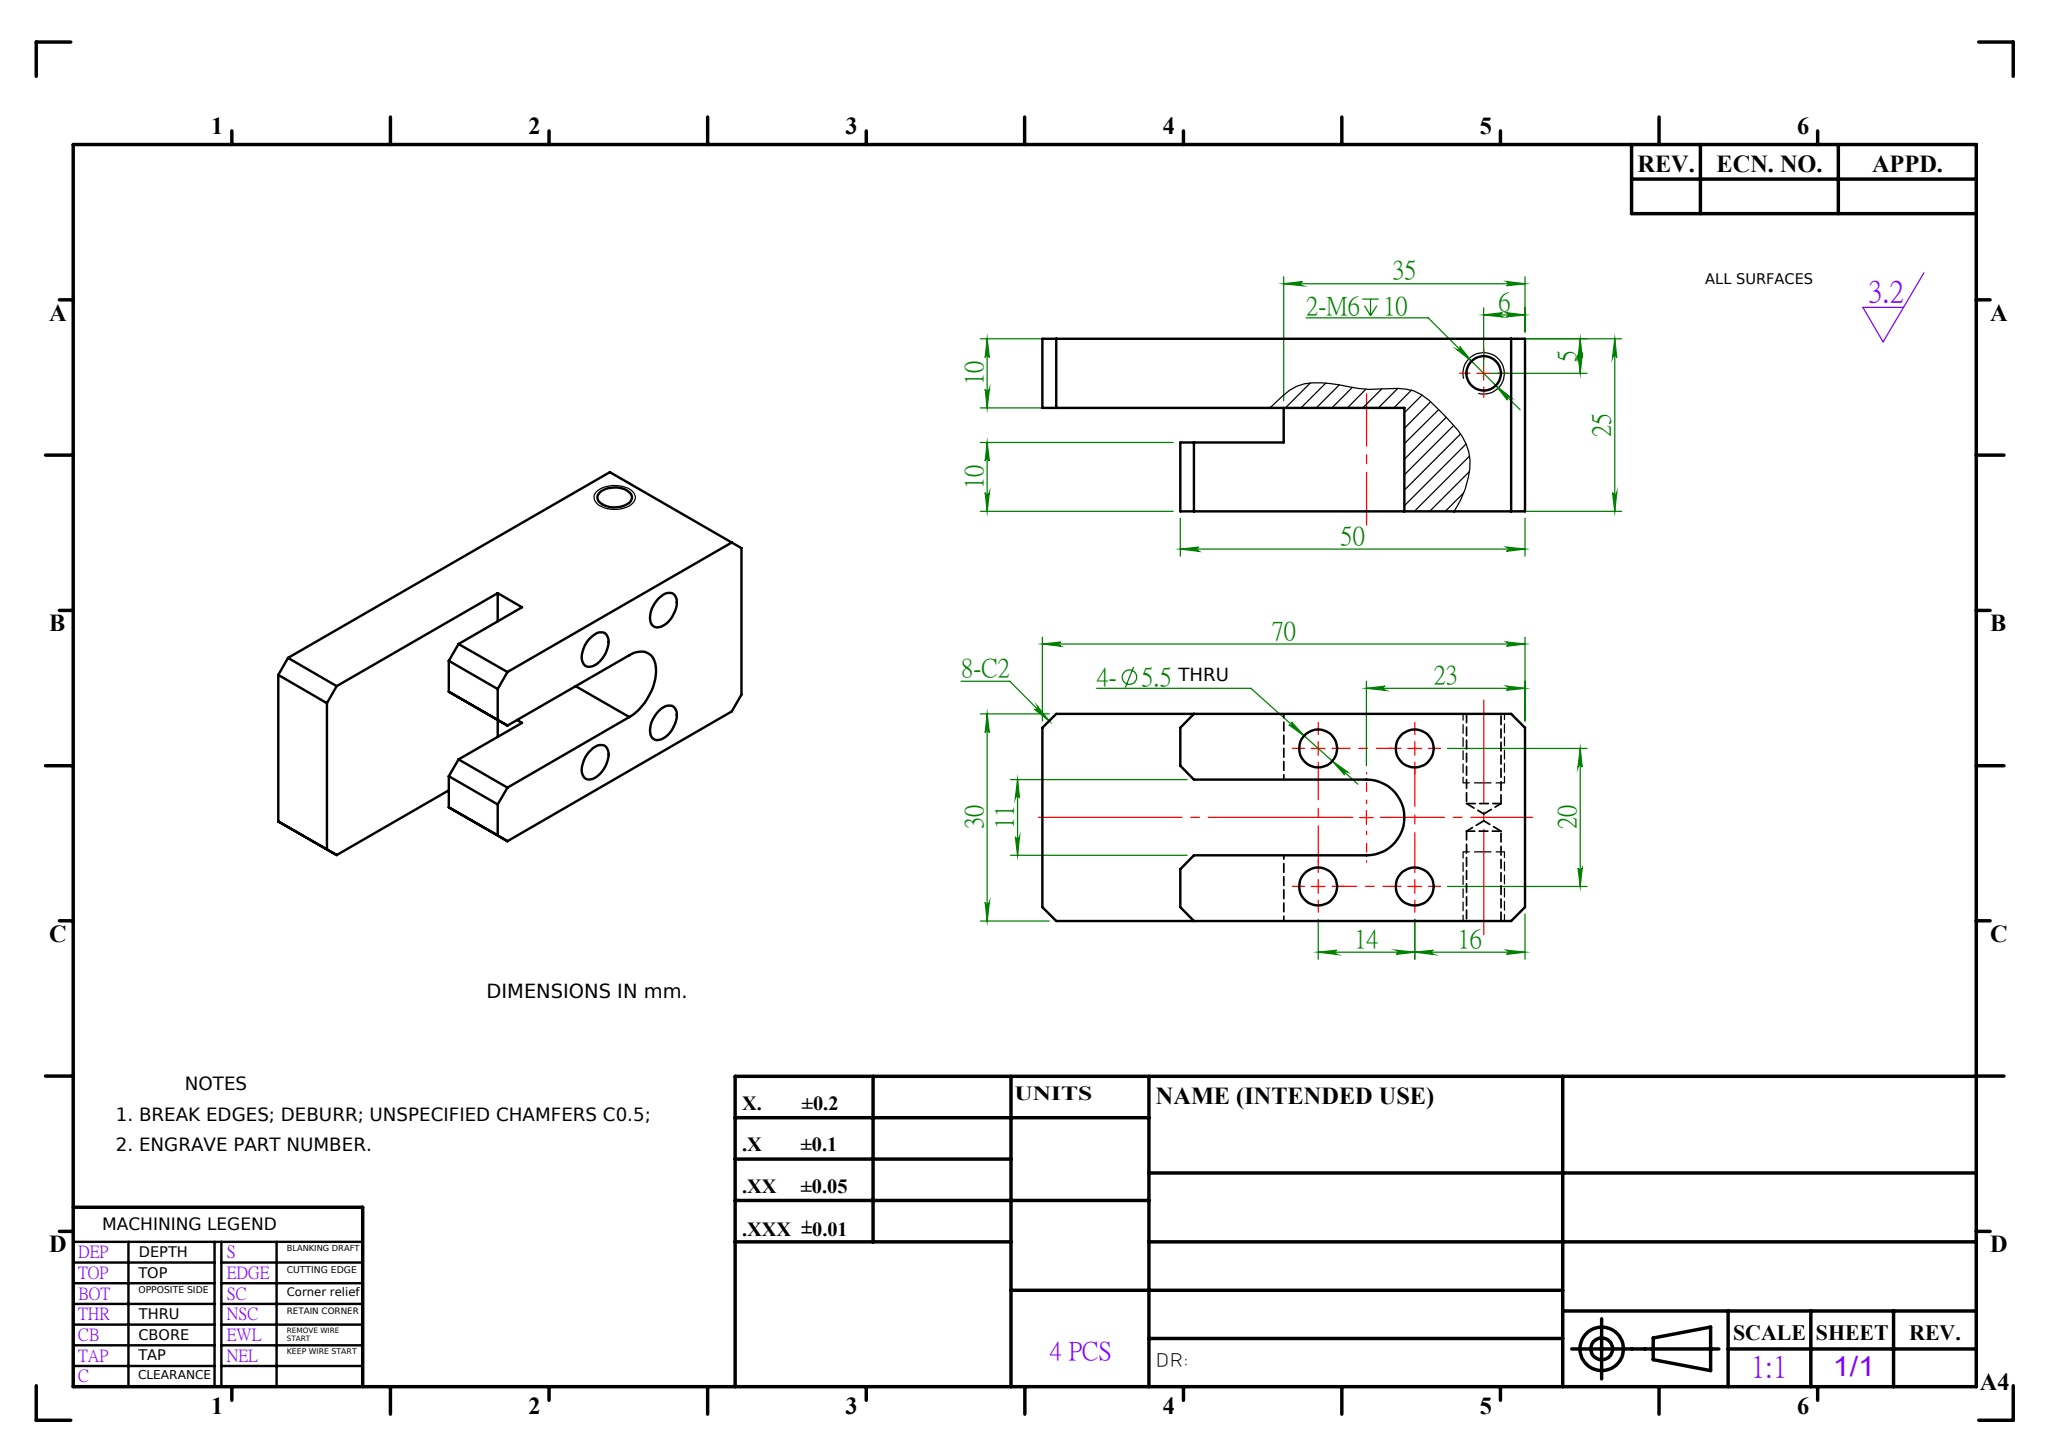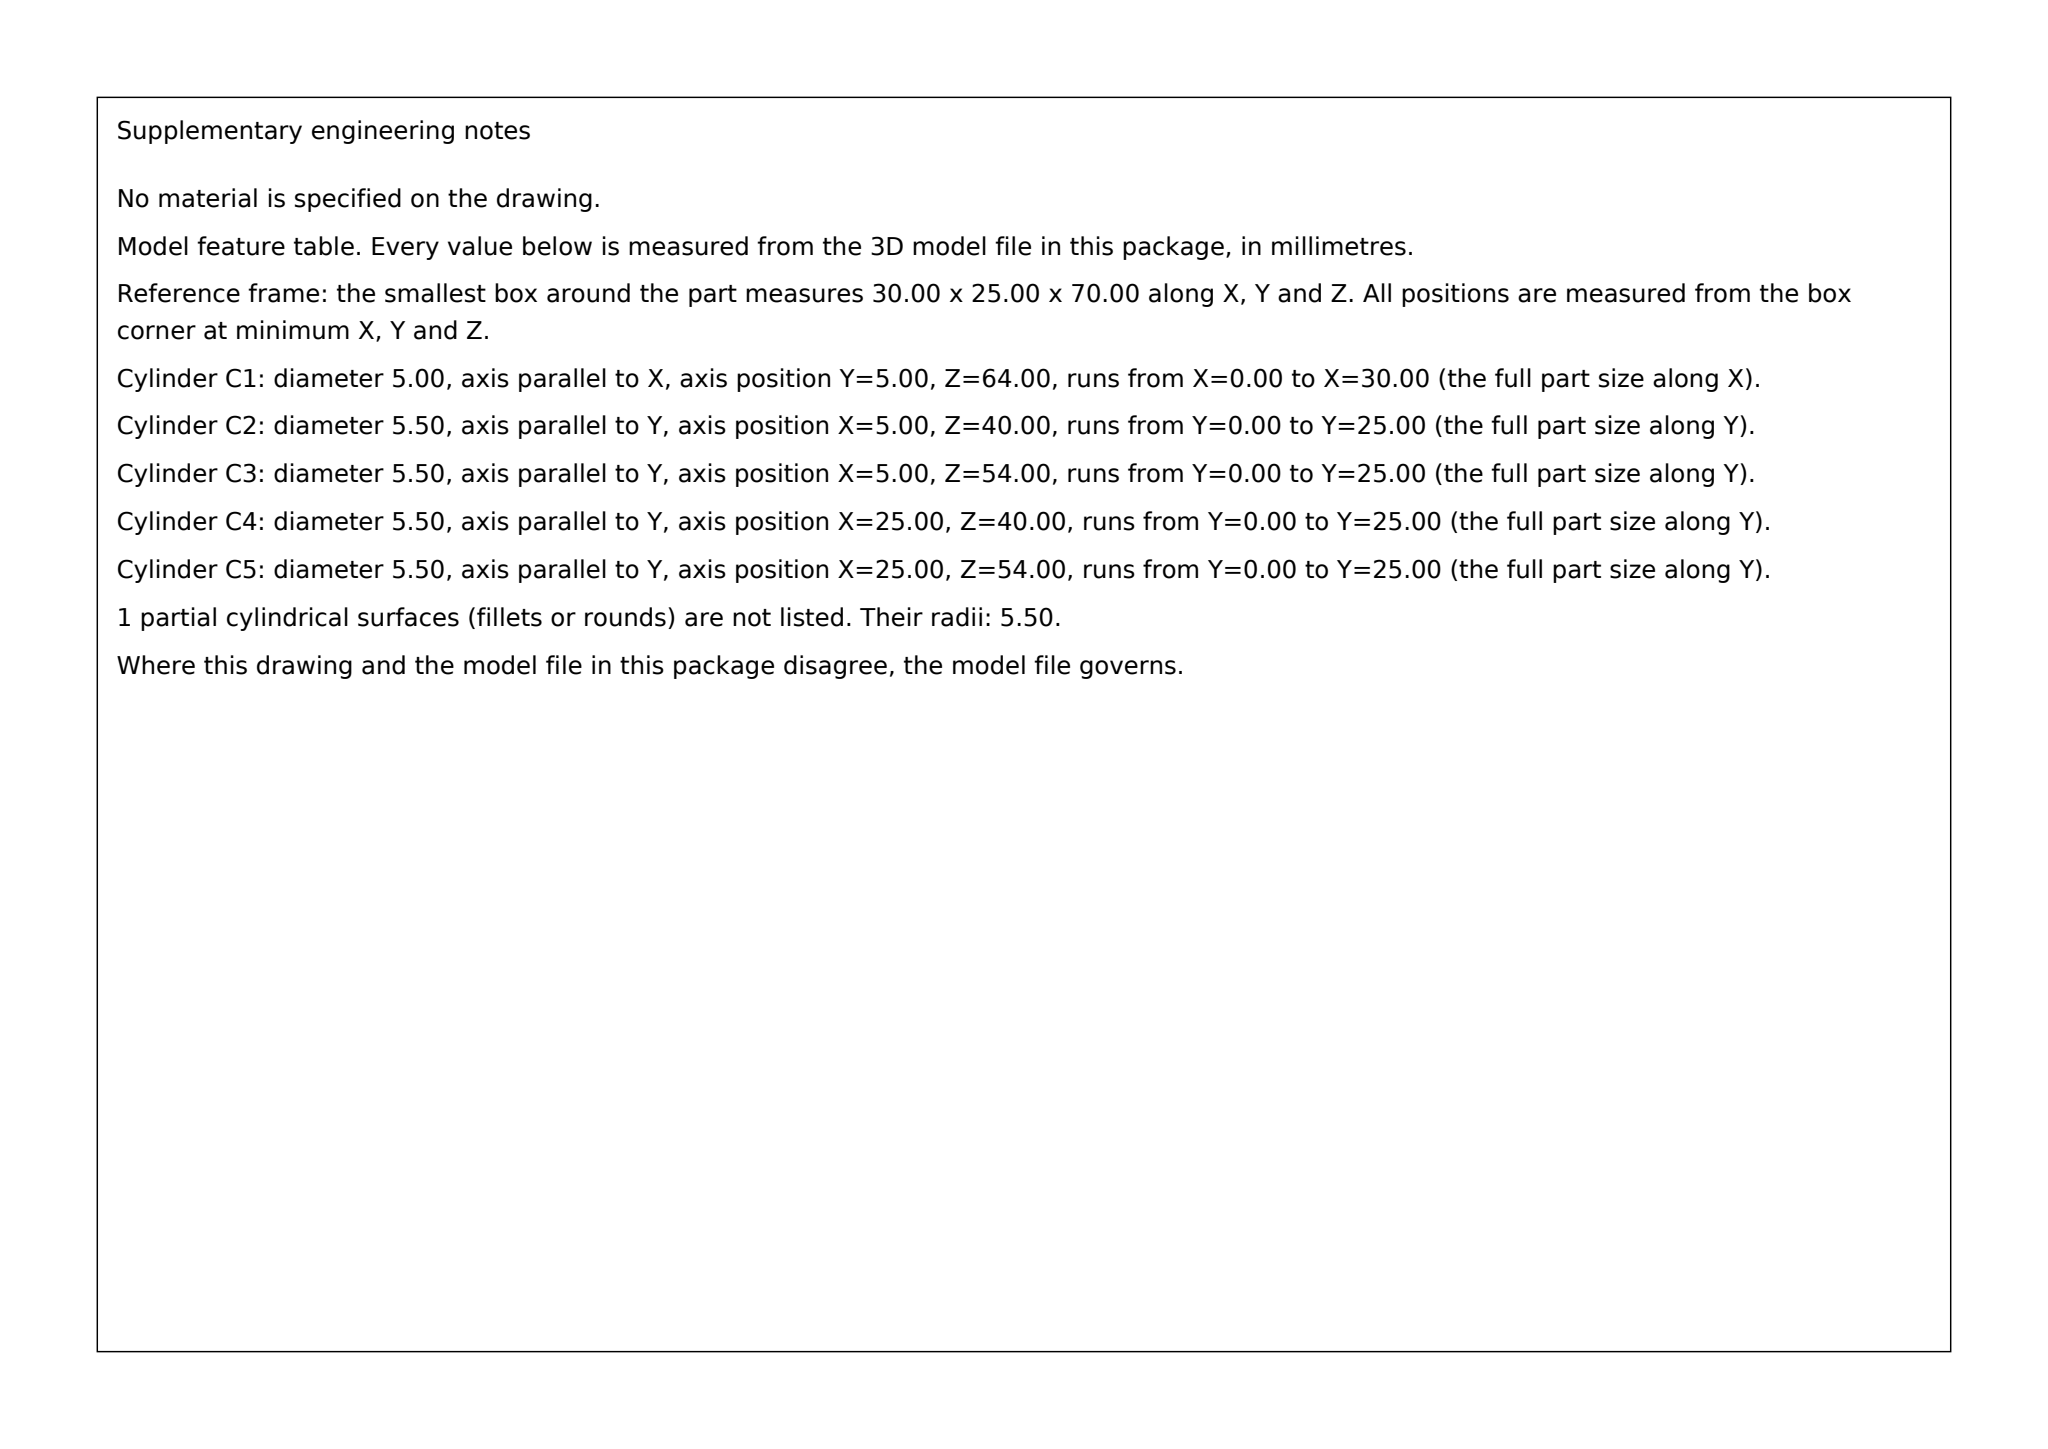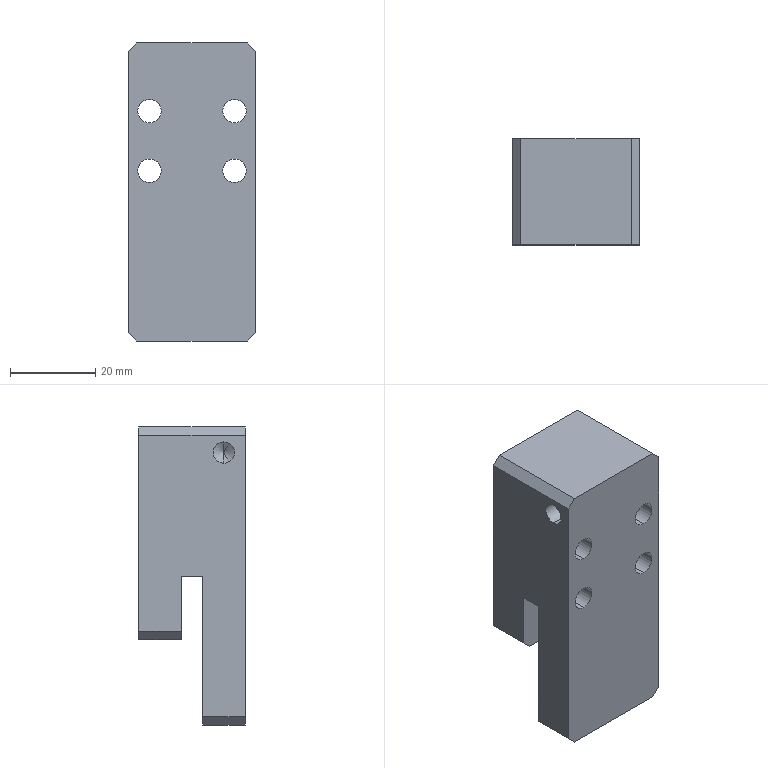Part | SolidWorks | mm | 1 solid | 41 faces | box 30 x 25 x 70 mm | volume 33781 mm3 | plane 23 | cylinder 14 | cone 4 | commonest cylinder face diameters 5.5 x8 5 x4 11 x2
build123d program:
from build123d import *

# Parameters (mm, degrees)
SKETCH1_W           = 30
SKETCH1_H           = 70
BOSS_EXTRUDE1_DEPTH = 12.5
CUT_EXTRUDE1_DEPTH  = 48.762
CUT_EXTRUDE3_DEPTH  = 15
CHAMFER1_SIZE       = 2
SKETCH6_R           = 2.75
CUT_EXTRUDE4_DEPTH  = 46.552


with BuildPart() as part:
    # Sketch1 → Boss-Extrude1 (new, symmetric)
    with BuildSketch(Plane(origin=(0, 0, 0), x_dir=(1, 0, 0), z_dir=(0, 1, 0))):
        Rectangle(SKETCH1_W, SKETCH1_H)
    extrude(amount=BOSS_EXTRUDE1_DEPTH, both=True)

    # Sketch2 → Cut-Extrude1 (cut, through all)
    with BuildSketch(Plane.ZY.offset(15)):
        Polygon((-35, 12.5), (-35, -2.5), (0, -2.5), (0, 2.5), (-15, 2.5), (-15, 12.5), align=None)
    extrude(amount=-CUT_EXTRUDE1_DEPTH, mode=Mode.SUBTRACT)

    # Sketch5 → Cut-Extrude3 (cut)
    with BuildSketch(Plane(origin=(0, 12.5, 0), x_dir=(1, 0, 0), z_dir=(0, 1, 0))):
        with BuildLine():
            Line((5.5, 18), (5.5, -12))
            ThreePointArc((5.5, -12), (0, -17.5), (-5.5, -12))
            Line((-5.5, -12), (-5.5, 18))
            ThreePointArc((-5.5, 18), (0, 23.5), (5.5, 18))
        make_face()
    extrude(amount=-CUT_EXTRUDE3_DEPTH, mode=Mode.SUBTRACT)

    # Chamfer1
    chamfer1_edges = [part.edges().sort_by_distance(p)[0] for p in [
        (-15, -7.5, -35),
        (15, -7.5, -35),
        (15, 7.5, -15),
        (-15, 7.5, -15),
        (5.5, 7.5, -15),
        (-5.5, 7.5, -15),
        (15, 0, 35),
        (-15, 0, 35),
    ]]
    chamfer(chamfer1_edges, length=CHAMFER1_SIZE)

    # Sketch6 → Cut-Extrude4 (cut, through all)
    with BuildSketch(Plane(origin=(0, 12.5, 0), x_dir=(1, 0, 0), z_dir=(0, 1, 0))):
        with Locations(Location((10, -5, 0), (0, 0, 270))):
            Circle(SKETCH6_R)
        with Locations(Location((-10, -5, 0), (0, 0, 270))):
            Circle(SKETCH6_R)
        with Locations(Location((-10, -19, 0), (0, 0, 270))):
            Circle(SKETCH6_R)
        with Locations(Location((10, -19, 0), (0, 0, 270))):
            Circle(SKETCH6_R)
    extrude(amount=-CUT_EXTRUDE4_DEPTH, mode=Mode.SUBTRACT)

    # Sketch7 → M6 Tapped Hole1 (revolve, cut)
    with BuildSketch(Plane(origin=(15, -7.5, 29), x_dir=(0, 0, -1), z_dir=(0, 1, 0))):
        Polygon((0, 0), (0, 14.502), (2.5, 13), (2.5, 0), align=None)
    m6_tapped_hole1 = revolve(axis=Axis((21.35, -7.5, 29), (-1, 0, 0)), mode=Mode.SUBTRACT)

    # Mirror1: M6 Tapped Hole1 across plane
    add(m6_tapped_hole1.mirror(Plane(origin=(0, 0, 0), x_dir=(0, 0, 1), z_dir=(1, 0, 0))), mode=Mode.SUBTRACT)


solid = part.part